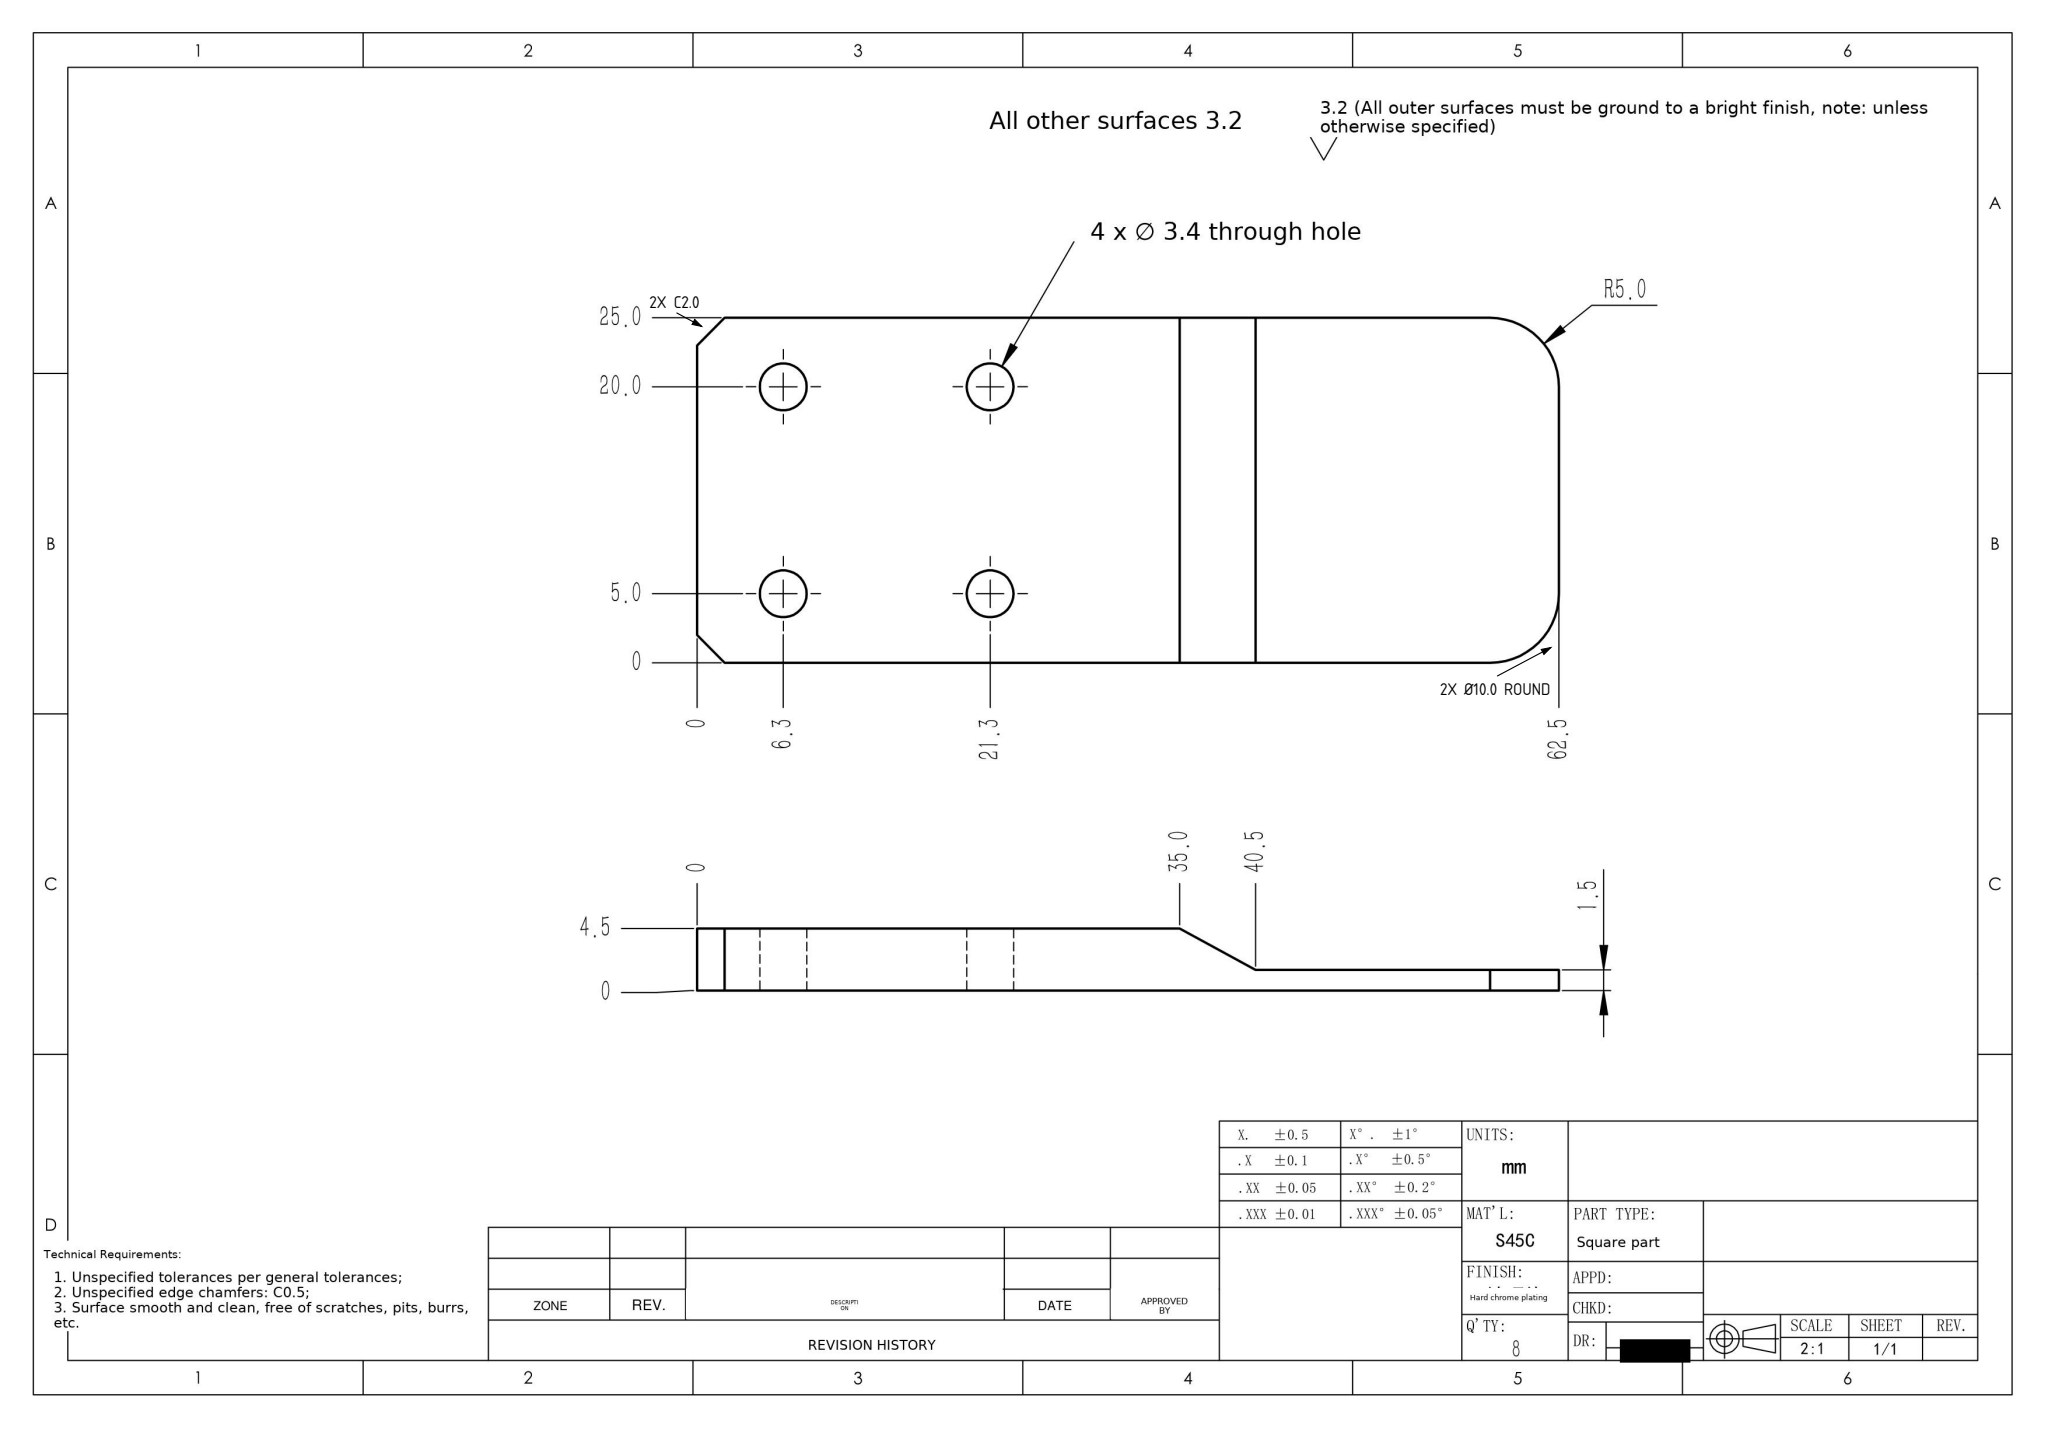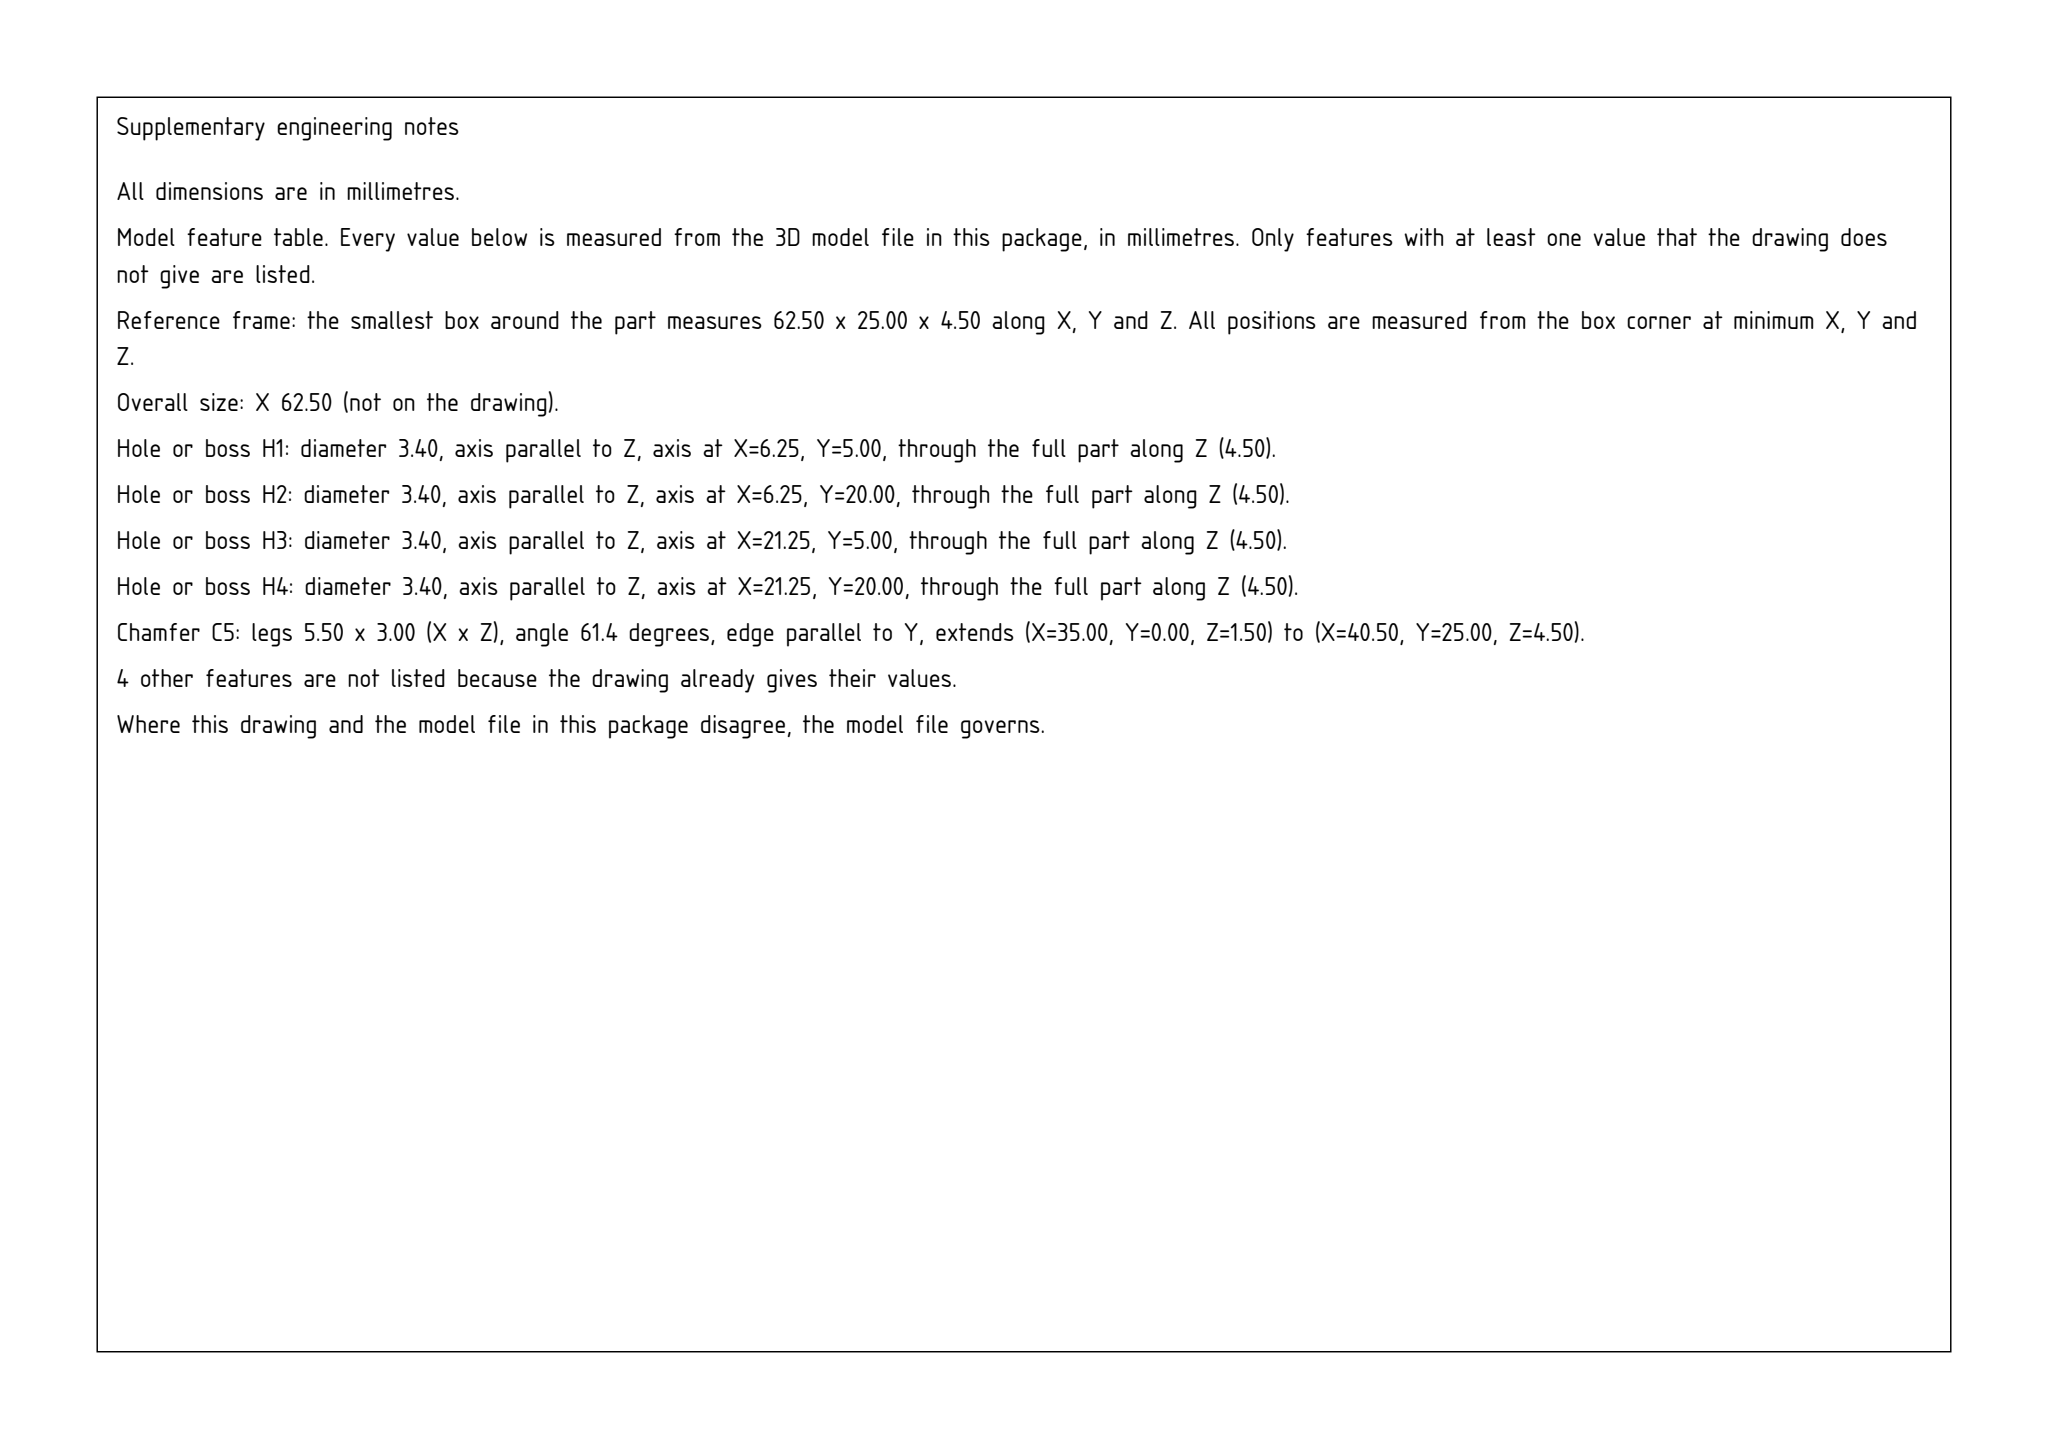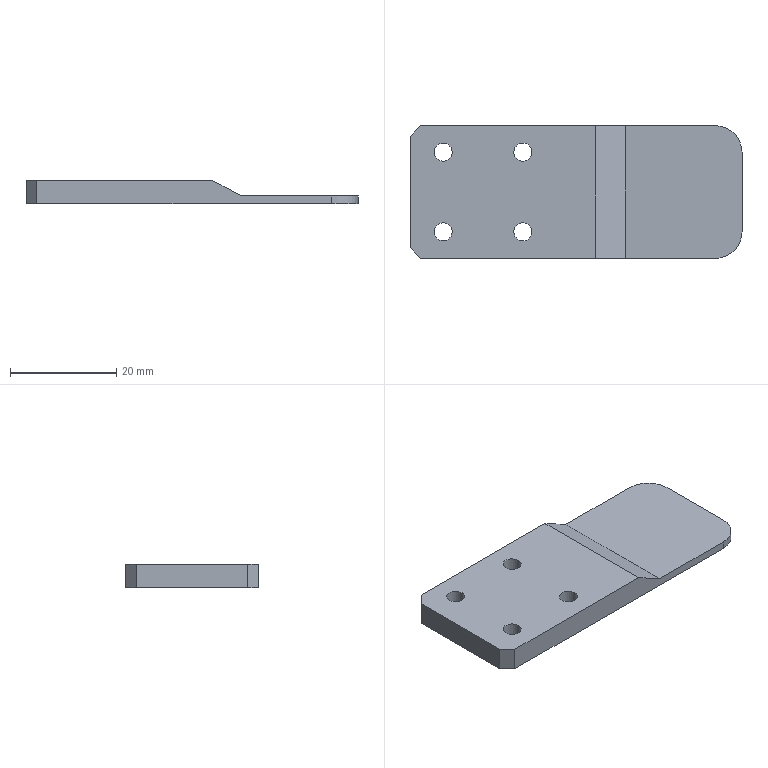Part | SolidWorks | mm | material S45C | 1 solid | 20 faces | box 62.5 x 25 x 4.5 mm | volume 4977 mm3 | cylinder 10 | plane 10 | commonest cylinder face diameters 3.4 x8 10 x2
Drawing notes:
2X Ø10.0 feature through the 1.5 thk end section, axes normal to the top face, centers at X=57.5 from the left end face and Y=5.0 and Y=20.0 from the bottom edge. | from the solid: cylinders [10.0, axis z, pos (57.5, 5.0) and (57.5, 20.0), length 1.5]
2X CHAMFER 2.0 X 45° ON LEFT END VERTICAL CORNERS (AT X=0 FACE, AT Y=0 AND Y=25.0 EDGES), FULL 4.5 THICKNESS | from the solid: inclined_planes: two faces at 45.0/45.0/90.0 deg, bbox_from [0.0,0.0,0.0] and [0.0,23.0,0.0], size [2.0,2.0,4.5]; x=0 plane extent y 2.0-23.0 confirms 2.0 legs
build123d program:
from build123d import *

# Parameters (mm, degrees)
SKETCH2_W            = 62.5
SKETCH2_H            = 25
BOSS_EXTRUDE1_DEPTH  = 4.5
CUT_EXTRUDE1_DEPTH   = 41.272
M3_CLEARANCE_HOLE1_D = 3.4
FILLET1_R            = 5
CHAMFER1_SIZE        = 2


with BuildPart() as part:
    # Sketch2 → Boss-Extrude1 (new body)
    with BuildSketch(Plane.XY):
        Rectangle(SKETCH2_W, SKETCH2_H)
    extrude(amount=BOSS_EXTRUDE1_DEPTH)

    # Sketch3 → Cut-Extrude1 (cut, through all)
    with BuildSketch(Plane.XZ.offset(12.5)):
        Polygon((31.25, 1.5), (9.25, 1.5), (3.75, 4.5), (31.25, 4.5), align=None)
    extrude(amount=-CUT_EXTRUDE1_DEPTH, mode=Mode.SUBTRACT)

    # M3 Clearance Hole1 (through all)
    with Locations(Plane(origin=(0, 0, 0), x_dir=(-1, 0, 0), z_dir=(0, 0, -1))):
        with Locations((10, -7.5), (10, 7.5), (25, 7.5), (25, -7.5)):
            Hole(M3_CLEARANCE_HOLE1_D / 2)

    # Fillet1
    fillet1_edges = [part.edges().sort_by_distance(p)[0] for p in [
        (31.25, -12.5, 0.75),
        (31.25, 12.5, 0.75),
    ]]
    fillet(fillet1_edges, radius=FILLET1_R)

    # Chamfer1
    chamfer1_edges = [part.edges().sort_by_distance(p)[0] for p in [
        (-31.25, -12.5, 2.25),
        (-31.25, 12.5, 2.25),
    ]]
    chamfer(chamfer1_edges, length=CHAMFER1_SIZE)


solid = part.part
STEP:
#1=CARTESIAN_POINT('',(-8.3,-7.5,4.5));
#2=VERTEX_POINT('',#1);
#3=CARTESIAN_POINT('',(-11.7,-7.5,4.5));
#4=VERTEX_POINT('',#3);
#5=CARTESIAN_POINT('',(-10.,-7.5,4.5));
#6=DIRECTION('',(0.,0.,-1.));
#7=DIRECTION('',(-1.,0.,0.));
#8=AXIS2_PLACEMENT_3D('',#5,#6,#7);
#9=CIRCLE('',#8,1.7);
#10=EDGE_CURVE('',#2,#4,#9,.T.);
#11=ORIENTED_EDGE('',*,*,#10,.F.);
#12=CARTESIAN_POINT('',(-8.3,-7.5,-0.));
#13=VERTEX_POINT('',#12);
#14=CARTESIAN_POINT('',(-8.3,-7.5,0.));
#15=DIRECTION('',(0.,0.,-1.));
#16=VECTOR('',#15,1000.);
#17=LINE('',#14,#16);
#18=EDGE_CURVE('',#2,#13,#17,.T.);
#19=ORIENTED_EDGE('',*,*,#18,.T.);
#20=CARTESIAN_POINT('',(-11.7,-7.5,-0.));
#21=VERTEX_POINT('',#20);
#22=CARTESIAN_POINT('',(-10.,-7.5,-0.));
#23=DIRECTION('',(0.,0.,-1.));
#24=DIRECTION('',(-1.,0.,0.));
#25=AXIS2_PLACEMENT_3D('',#22,#23,#24);
#26=CIRCLE('',#25,1.7);
#27=EDGE_CURVE('',#13,#21,#26,.T.);
#28=ORIENTED_EDGE('',*,*,#27,.T.);
#29=CARTESIAN_POINT('',(-11.7,-7.5,0.));
#30=DIRECTION('',(0.,0.,-1.));
#31=VECTOR('',#30,1000.);
#32=LINE('',#29,#31);
#33=EDGE_CURVE('',#4,#21,#32,.T.);
#34=ORIENTED_EDGE('',*,*,#33,.F.);
#35=EDGE_LOOP('',(#11,#19,#28,#34));
#36=FACE_OUTER_BOUND('',#35,.T.);
#37=CARTESIAN_POINT('',(-10.,-7.5,0.));
#38=DIRECTION('',(0.,0.,-1.));
#39=DIRECTION('',(-1.,0.,0.));
#40=AXIS2_PLACEMENT_3D('',#37,#38,#39);
#41=CYLINDRICAL_SURFACE('',#40,1.7);
#42=ADVANCED_FACE('',(#36),#41,.F.);
#43=CARTESIAN_POINT('',(-8.3,7.5,4.5));
#44=VERTEX_POINT('',#43);
#45=CARTESIAN_POINT('',(-11.7,7.5,4.5));
#46=VERTEX_POINT('',#45);
#47=CARTESIAN_POINT('',(-10.,7.5,4.5));
#48=DIRECTION('',(0.,0.,-1.));
#49=DIRECTION('',(-1.,0.,0.));
#50=AXIS2_PLACEMENT_3D('',#47,#48,#49);
#51=CIRCLE('',#50,1.7);
#52=EDGE_CURVE('',#44,#46,#51,.T.);
#53=ORIENTED_EDGE('',*,*,#52,.F.);
#54=CARTESIAN_POINT('',(-8.3,7.5,-0.));
#55=VERTEX_POINT('',#54);
#56=CARTESIAN_POINT('',(-8.3,7.5,0.));
#57=DIRECTION('',(0.,0.,-1.));
#58=VECTOR('',#57,1000.);
#59=LINE('',#56,#58);
#60=EDGE_CURVE('',#44,#55,#59,.T.);
#61=ORIENTED_EDGE('',*,*,#60,.T.);
#62=CARTESIAN_POINT('',(-11.7,7.5,-0.));
#63=VERTEX_POINT('',#62);
#64=CARTESIAN_POINT('',(-10.,7.5,-0.));
#65=DIRECTION('',(0.,0.,-1.));
#66=DIRECTION('',(-1.,0.,0.));
#67=AXIS2_PLACEMENT_3D('',#64,#65,#66);
#68=CIRCLE('',#67,1.7);
#69=EDGE_CURVE('',#55,#63,#68,.T.);
#70=ORIENTED_EDGE('',*,*,#69,.T.);
#71=CARTESIAN_POINT('',(-11.7,7.5,0.));
#72=DIRECTION('',(0.,0.,-1.));
#73=VECTOR('',#72,1000.);
#74=LINE('',#71,#73);
#75=EDGE_CURVE('',#46,#63,#74,.T.);
#76=ORIENTED_EDGE('',*,*,#75,.F.);
#77=EDGE_LOOP('',(#53,#61,#70,#76));
#78=FACE_OUTER_BOUND('',#77,.T.);
#79=CARTESIAN_POINT('',(-10.,7.5,0.));
#80=DIRECTION('',(0.,0.,-1.));
#81=DIRECTION('',(-1.,0.,0.));
#82=AXIS2_PLACEMENT_3D('',#79,#80,#81);
#83=CYLINDRICAL_SURFACE('',#82,1.7);
#84=ADVANCED_FACE('',(#78),#83,.F.);
#85=CARTESIAN_POINT('',(-23.3,7.5,4.5));
#86=VERTEX_POINT('',#85);
#87=CARTESIAN_POINT('',(-26.7,7.5,4.5));
#88=VERTEX_POINT('',#87);
#89=CARTESIAN_POINT('',(-25.,7.5,4.5));
#90=DIRECTION('',(0.,0.,-1.));
#91=DIRECTION('',(-1.,0.,0.));
#92=AXIS2_PLACEMENT_3D('',#89,#90,#91);
#93=CIRCLE('',#92,1.7);
#94=EDGE_CURVE('',#86,#88,#93,.T.);
#95=ORIENTED_EDGE('',*,*,#94,.F.);
#96=CARTESIAN_POINT('',(-23.3,7.5,-0.));
#97=VERTEX_POINT('',#96);
#98=CARTESIAN_POINT('',(-23.3,7.5,0.));
#99=DIRECTION('',(0.,0.,-1.));
#100=VECTOR('',#99,1000.);
#101=LINE('',#98,#100);
#102=EDGE_CURVE('',#86,#97,#101,.T.);
#103=ORIENTED_EDGE('',*,*,#102,.T.);
#104=CARTESIAN_POINT('',(-26.7,7.5,-0.));
#105=VERTEX_POINT('',#104);
#106=CARTESIAN_POINT('',(-25.,7.5,-0.));
#107=DIRECTION('',(0.,0.,-1.));
#108=DIRECTION('',(-1.,0.,0.));
#109=AXIS2_PLACEMENT_3D('',#106,#107,#108);
#110=CIRCLE('',#109,1.7);
#111=EDGE_CURVE('',#97,#105,#110,.T.);
#112=ORIENTED_EDGE('',*,*,#111,.T.);
#113=CARTESIAN_POINT('',(-26.7,7.5,0.));
#114=DIRECTION('',(0.,0.,-1.));
#115=VECTOR('',#114,1000.);
#116=LINE('',#113,#115);
#117=EDGE_CURVE('',#88,#105,#116,.T.);
#118=ORIENTED_EDGE('',*,*,#117,.F.);
#119=EDGE_LOOP('',(#95,#103,#112,#118));
#120=FACE_OUTER_BOUND('',#119,.T.);
#121=CARTESIAN_POINT('',(-25.,7.5,0.));
#122=DIRECTION('',(0.,0.,-1.));
#123=DIRECTION('',(-1.,0.,0.));
#124=AXIS2_PLACEMENT_3D('',#121,#122,#123);
#125=CYLINDRICAL_SURFACE('',#124,1.7);
#126=ADVANCED_FACE('',(#120),#125,.F.);
#127=CARTESIAN_POINT('',(-23.3,-7.5,4.5));
#128=VERTEX_POINT('',#127);
#129=CARTESIAN_POINT('',(-26.7,-7.5,4.5));
#130=VERTEX_POINT('',#129);
#131=CARTESIAN_POINT('',(-25.,-7.5,4.5));
#132=DIRECTION('',(0.,0.,-1.));
#133=DIRECTION('',(-1.,0.,0.));
#134=AXIS2_PLACEMENT_3D('',#131,#132,#133);
#135=CIRCLE('',#134,1.7);
#136=EDGE_CURVE('',#128,#130,#135,.T.);
#137=ORIENTED_EDGE('',*,*,#136,.F.);
#138=CARTESIAN_POINT('',(-23.3,-7.5,-0.));
#139=VERTEX_POINT('',#138);
#140=CARTESIAN_POINT('',(-23.3,-7.5,0.));
#141=DIRECTION('',(0.,0.,-1.));
#142=VECTOR('',#141,1000.);
#143=LINE('',#140,#142);
#144=EDGE_CURVE('',#128,#139,#143,.T.);
#145=ORIENTED_EDGE('',*,*,#144,.T.);
#146=CARTESIAN_POINT('',(-26.7,-7.5,-0.));
#147=VERTEX_POINT('',#146);
#148=CARTESIAN_POINT('',(-25.,-7.5,-0.));
#149=DIRECTION('',(0.,0.,-1.));
#150=DIRECTION('',(-1.,0.,0.));
#151=AXIS2_PLACEMENT_3D('',#148,#149,#150);
#152=CIRCLE('',#151,1.7);
#153=EDGE_CURVE('',#139,#147,#152,.T.);
#154=ORIENTED_EDGE('',*,*,#153,.T.);
#155=CARTESIAN_POINT('',(-26.7,-7.5,0.));
#156=DIRECTION('',(0.,0.,-1.));
#157=VECTOR('',#156,1000.);
#158=LINE('',#155,#157);
#159=EDGE_CURVE('',#130,#147,#158,.T.);
#160=ORIENTED_EDGE('',*,*,#159,.F.);
#161=EDGE_LOOP('',(#137,#145,#154,#160));
#162=FACE_OUTER_BOUND('',#161,.T.);
#163=CARTESIAN_POINT('',(-25.,-7.5,0.));
#164=DIRECTION('',(0.,0.,-1.));
#165=DIRECTION('',(-1.,0.,0.));
#166=AXIS2_PLACEMENT_3D('',#163,#164,#165);
#167=CYLINDRICAL_SURFACE('',#166,1.7);
#168=ADVANCED_FACE('',(#162),#167,.F.);
#169=CARTESIAN_POINT('',(31.25,7.5,1.5));
#170=VERTEX_POINT('',#169);
#171=CARTESIAN_POINT('',(31.25,-7.5,1.5));
#172=VERTEX_POINT('',#171);
#173=CARTESIAN_POINT('',(31.25,12.5,1.5));
#174=DIRECTION('',(0.,-1.,0.));
#175=VECTOR('',#174,1000.);
#176=LINE('',#173,#175);
#177=EDGE_CURVE('',#170,#172,#176,.T.);
#178=ORIENTED_EDGE('',*,*,#177,.T.);
#179=CARTESIAN_POINT('',(31.25,-7.5,0.));
#180=VERTEX_POINT('',#179);
#181=CARTESIAN_POINT('',(31.25,-7.5,4.5));
#182=DIRECTION('',(0.,0.,-1.));
#183=VECTOR('',#182,1000.);
#184=LINE('',#181,#183);
#185=EDGE_CURVE('',#172,#180,#184,.T.);
#186=ORIENTED_EDGE('',*,*,#185,.T.);
#187=CARTESIAN_POINT('',(31.25,7.5,0.));
#188=VERTEX_POINT('',#187);
#189=CARTESIAN_POINT('',(31.25,12.5,0.));
#190=DIRECTION('',(0.,1.,0.));
#191=VECTOR('',#190,1000.);
#192=LINE('',#189,#191);
#193=EDGE_CURVE('',#180,#188,#192,.T.);
#194=ORIENTED_EDGE('',*,*,#193,.T.);
#195=CARTESIAN_POINT('',(31.25,7.5,4.5));
#196=DIRECTION('',(0.,0.,1.));
#197=VECTOR('',#196,1000.);
#198=LINE('',#195,#197);
#199=EDGE_CURVE('',#188,#170,#198,.T.);
#200=ORIENTED_EDGE('',*,*,#199,.T.);
#201=EDGE_LOOP('',(#178,#186,#194,#200));
#202=FACE_OUTER_BOUND('',#201,.T.);
#203=CARTESIAN_POINT('',(31.25,12.5,4.5));
#204=DIRECTION('',(-1.,0.,0.));
#205=DIRECTION('',(0.,0.,1.));
#206=AXIS2_PLACEMENT_3D('',#203,#204,#205);
#207=PLANE('',#206);
#208=ADVANCED_FACE('',(#202),#207,.F.);
#209=CARTESIAN_POINT('',(26.25,12.5,0.));
#210=VERTEX_POINT('',#209);
#211=CARTESIAN_POINT('',(-29.25,12.5,0.));
#212=VERTEX_POINT('',#211);
#213=CARTESIAN_POINT('',(-31.25,12.5,0.));
#214=DIRECTION('',(-1.,0.,0.));
#215=VECTOR('',#214,1000.);
#216=LINE('',#213,#215);
#217=EDGE_CURVE('',#210,#212,#216,.T.);
#218=ORIENTED_EDGE('',*,*,#217,.T.);
#219=CARTESIAN_POINT('',(-29.25,12.5,4.5));
#220=VERTEX_POINT('',#219);
#221=CARTESIAN_POINT('',(-29.25,12.5,4.5));
#222=DIRECTION('',(0.,0.,1.));
#223=VECTOR('',#222,1000.);
#224=LINE('',#221,#223);
#225=EDGE_CURVE('',#212,#220,#224,.T.);
#226=ORIENTED_EDGE('',*,*,#225,.T.);
#227=CARTESIAN_POINT('',(3.75,12.5,4.5));
#228=VERTEX_POINT('',#227);
#229=CARTESIAN_POINT('',(-31.25,12.5,4.5));
#230=DIRECTION('',(-1.,0.,0.));
#231=VECTOR('',#230,1000.);
#232=LINE('',#229,#231);
#233=EDGE_CURVE('',#228,#220,#232,.T.);
#234=ORIENTED_EDGE('',*,*,#233,.F.);
#235=CARTESIAN_POINT('',(9.25,12.5,1.5));
#236=VERTEX_POINT('',#235);
#237=CARTESIAN_POINT('',(9.25,12.5,1.5));
#238=DIRECTION('',(0.8779,0.,-0.4789));
#239=VECTOR('',#238,1000.);
#240=LINE('',#237,#239);
#241=EDGE_CURVE('',#228,#236,#240,.T.);
#242=ORIENTED_EDGE('',*,*,#241,.T.);
#243=CARTESIAN_POINT('',(26.25,12.5,1.5));
#244=VERTEX_POINT('',#243);
#245=CARTESIAN_POINT('',(31.25,12.5,1.5));
#246=DIRECTION('',(1.,0.,0.));
#247=VECTOR('',#246,1000.);
#248=LINE('',#245,#247);
#249=EDGE_CURVE('',#236,#244,#248,.T.);
#250=ORIENTED_EDGE('',*,*,#249,.T.);
#251=CARTESIAN_POINT('',(26.25,12.5,4.5));
#252=DIRECTION('',(0.,0.,-1.));
#253=VECTOR('',#252,1000.);
#254=LINE('',#251,#253);
#255=EDGE_CURVE('',#244,#210,#254,.T.);
#256=ORIENTED_EDGE('',*,*,#255,.T.);
#257=EDGE_LOOP('',(#218,#226,#234,#242,#250,#256));
#258=FACE_OUTER_BOUND('',#257,.T.);
#259=CARTESIAN_POINT('',(-31.25,12.5,4.5));
#260=DIRECTION('',(0.,-1.,0.));
#261=DIRECTION('',(0.,0.,-1.));
#262=AXIS2_PLACEMENT_3D('',#259,#260,#261);
#263=PLANE('',#262);
#264=ADVANCED_FACE('',(#258),#263,.F.);
#265=CARTESIAN_POINT('',(-31.25,10.5,4.5));
#266=VERTEX_POINT('',#265);
#267=CARTESIAN_POINT('',(-31.25,-10.5,4.5));
#268=VERTEX_POINT('',#267);
#269=CARTESIAN_POINT('',(-31.25,12.5,4.5));
#270=DIRECTION('',(0.,-1.,0.));
#271=VECTOR('',#270,1000.);
#272=LINE('',#269,#271);
#273=EDGE_CURVE('',#266,#268,#272,.T.);
#274=ORIENTED_EDGE('',*,*,#273,.F.);
#275=CARTESIAN_POINT('',(-31.25,10.5,0.));
#276=VERTEX_POINT('',#275);
#277=CARTESIAN_POINT('',(-31.25,10.5,4.5));
#278=DIRECTION('',(0.,0.,-1.));
#279=VECTOR('',#278,1000.);
#280=LINE('',#277,#279);
#281=EDGE_CURVE('',#266,#276,#280,.T.);
#282=ORIENTED_EDGE('',*,*,#281,.T.);
#283=CARTESIAN_POINT('',(-31.25,-10.5,0.));
#284=VERTEX_POINT('',#283);
#285=CARTESIAN_POINT('',(-31.25,12.5,0.));
#286=DIRECTION('',(0.,-1.,0.));
#287=VECTOR('',#286,1000.);
#288=LINE('',#285,#287);
#289=EDGE_CURVE('',#276,#284,#288,.T.);
#290=ORIENTED_EDGE('',*,*,#289,.T.);
#291=CARTESIAN_POINT('',(-31.25,-10.5,4.5));
#292=DIRECTION('',(0.,0.,1.));
#293=VECTOR('',#292,1000.);
#294=LINE('',#291,#293);
#295=EDGE_CURVE('',#284,#268,#294,.T.);
#296=ORIENTED_EDGE('',*,*,#295,.T.);
#297=EDGE_LOOP('',(#274,#282,#290,#296));
#298=FACE_OUTER_BOUND('',#297,.T.);
#299=CARTESIAN_POINT('',(-31.25,12.5,4.5));
#300=DIRECTION('',(1.,0.,0.));
#301=DIRECTION('',(-0.,1.,0.));
#302=AXIS2_PLACEMENT_3D('',#299,#300,#301);
#303=PLANE('',#302);
#304=ADVANCED_FACE('',(#298),#303,.F.);
#305=CARTESIAN_POINT('',(-29.25,-12.5,4.5));
#306=VERTEX_POINT('',#305);
#307=CARTESIAN_POINT('',(3.75,-12.5,4.5));
#308=VERTEX_POINT('',#307);
#309=CARTESIAN_POINT('',(-31.25,-12.5,4.5));
#310=DIRECTION('',(1.,0.,0.));
#311=VECTOR('',#310,1000.);
#312=LINE('',#309,#311);
#313=EDGE_CURVE('',#306,#308,#312,.T.);
#314=ORIENTED_EDGE('',*,*,#313,.F.);
#315=CARTESIAN_POINT('',(-29.25,-12.5,0.));
#316=VERTEX_POINT('',#315);
#317=CARTESIAN_POINT('',(-29.25,-12.5,4.5));
#318=DIRECTION('',(0.,0.,-1.));
#319=VECTOR('',#318,1000.);
#320=LINE('',#317,#319);
#321=EDGE_CURVE('',#306,#316,#320,.T.);
#322=ORIENTED_EDGE('',*,*,#321,.T.);
#323=CARTESIAN_POINT('',(26.25,-12.5,0.));
#324=VERTEX_POINT('',#323);
#325=CARTESIAN_POINT('',(-31.25,-12.5,0.));
#326=DIRECTION('',(1.,0.,0.));
#327=VECTOR('',#326,1000.);
#328=LINE('',#325,#327);
#329=EDGE_CURVE('',#316,#324,#328,.T.);
#330=ORIENTED_EDGE('',*,*,#329,.T.);
#331=CARTESIAN_POINT('',(26.25,-12.5,1.5));
#332=VERTEX_POINT('',#331);
#333=CARTESIAN_POINT('',(26.25,-12.5,4.5));
#334=DIRECTION('',(0.,0.,1.));
#335=VECTOR('',#334,1000.);
#336=LINE('',#333,#335);
#337=EDGE_CURVE('',#324,#332,#336,.T.);
#338=ORIENTED_EDGE('',*,*,#337,.T.);
#339=CARTESIAN_POINT('',(9.25,-12.5,1.5));
#340=VERTEX_POINT('',#339);
#341=CARTESIAN_POINT('',(31.25,-12.5,1.5));
#342=DIRECTION('',(1.,0.,0.));
#343=VECTOR('',#342,1000.);
#344=LINE('',#341,#343);
#345=EDGE_CURVE('',#340,#332,#344,.T.);
#346=ORIENTED_EDGE('',*,*,#345,.F.);
#347=CARTESIAN_POINT('',(9.25,-12.5,1.5));
#348=DIRECTION('',(0.8779,0.,-0.4789));
#349=VECTOR('',#348,1000.);
#350=LINE('',#347,#349);
#351=EDGE_CURVE('',#308,#340,#350,.T.);
#352=ORIENTED_EDGE('',*,*,#351,.F.);
#353=EDGE_LOOP('',(#314,#322,#330,#338,#346,#352));
#354=FACE_OUTER_BOUND('',#353,.T.);
#355=CARTESIAN_POINT('',(-31.25,-12.5,4.5));
#356=DIRECTION('',(0.,1.,0.));
#357=DIRECTION('',(0.,0.,1.));
#358=AXIS2_PLACEMENT_3D('',#355,#356,#357);
#359=PLANE('',#358);
#360=ADVANCED_FACE('',(#354),#359,.F.);
#361=CARTESIAN_POINT('',(-10.,-7.5,4.5));
#362=DIRECTION('',(0.,0.,-1.));
#363=DIRECTION('',(-1.,0.,0.));
#364=AXIS2_PLACEMENT_3D('',#361,#362,#363);
#365=CIRCLE('',#364,1.7);
#366=EDGE_CURVE('',#4,#2,#365,.T.);
#367=ORIENTED_EDGE('',*,*,#366,.T.);
#368=ORIENTED_EDGE('',*,*,#10,.T.);
#369=EDGE_LOOP('',(#367,#368));
#370=FACE_BOUND('',#369,.T.);
#371=CARTESIAN_POINT('',(-10.,7.5,4.5));
#372=DIRECTION('',(0.,0.,-1.));
#373=DIRECTION('',(-1.,0.,0.));
#374=AXIS2_PLACEMENT_3D('',#371,#372,#373);
#375=CIRCLE('',#374,1.7);
#376=EDGE_CURVE('',#46,#44,#375,.T.);
#377=ORIENTED_EDGE('',*,*,#376,.T.);
#378=ORIENTED_EDGE('',*,*,#52,.T.);
#379=EDGE_LOOP('',(#377,#378));
#380=FACE_BOUND('',#379,.T.);
#381=CARTESIAN_POINT('',(-25.,7.5,4.5));
#382=DIRECTION('',(0.,0.,-1.));
#383=DIRECTION('',(-1.,0.,0.));
#384=AXIS2_PLACEMENT_3D('',#381,#382,#383);
#385=CIRCLE('',#384,1.7);
#386=EDGE_CURVE('',#88,#86,#385,.T.);
#387=ORIENTED_EDGE('',*,*,#386,.T.);
#388=ORIENTED_EDGE('',*,*,#94,.T.);
#389=EDGE_LOOP('',(#387,#388));
#390=FACE_BOUND('',#389,.T.);
#391=CARTESIAN_POINT('',(-25.,-7.5,4.5));
#392=DIRECTION('',(0.,0.,-1.));
#393=DIRECTION('',(-1.,0.,0.));
#394=AXIS2_PLACEMENT_3D('',#391,#392,#393);
#395=CIRCLE('',#394,1.7);
#396=EDGE_CURVE('',#130,#128,#395,.T.);
#397=ORIENTED_EDGE('',*,*,#396,.T.);
#398=ORIENTED_EDGE('',*,*,#136,.T.);
#399=EDGE_LOOP('',(#397,#398));
#400=FACE_BOUND('',#399,.T.);
#401=ORIENTED_EDGE('',*,*,#233,.T.);
#402=CARTESIAN_POINT('',(-20.875,20.875,4.5));
#403=DIRECTION('',(-0.7071,-0.7071,0.));
#404=VECTOR('',#403,1000.);
#405=LINE('',#402,#404);
#406=EDGE_CURVE('',#220,#266,#405,.T.);
#407=ORIENTED_EDGE('',*,*,#406,.T.);
#408=ORIENTED_EDGE('',*,*,#273,.T.);
#409=CARTESIAN_POINT('',(-20.875,-20.875,4.5));
#410=DIRECTION('',(0.7071,-0.7071,0.));
#411=VECTOR('',#410,1000.);
#412=LINE('',#409,#411);
#413=EDGE_CURVE('',#268,#306,#412,.T.);
#414=ORIENTED_EDGE('',*,*,#413,.T.);
#415=ORIENTED_EDGE('',*,*,#313,.T.);
#416=CARTESIAN_POINT('',(3.75,12.5,4.5));
#417=DIRECTION('',(0.,-1.,0.));
#418=VECTOR('',#417,1000.);
#419=LINE('',#416,#418);
#420=EDGE_CURVE('',#228,#308,#419,.T.);
#421=ORIENTED_EDGE('',*,*,#420,.F.);
#422=EDGE_LOOP('',(#401,#407,#408,#414,#415,#421));
#423=FACE_OUTER_BOUND('',#422,.T.);
#424=CARTESIAN_POINT('',(0.,0.,4.5));
#425=DIRECTION('',(0.,0.,1.));
#426=DIRECTION('',(1.,0.,0.));
#427=AXIS2_PLACEMENT_3D('',#424,#425,#426);
#428=PLANE('',#427);
#429=ADVANCED_FACE('',(#370,#380,#390,#400,#423),#428,.T.);
#430=CARTESIAN_POINT('',(-10.,-7.5,-0.));
#431=DIRECTION('',(0.,0.,-1.));
#432=DIRECTION('',(-1.,0.,0.));
#433=AXIS2_PLACEMENT_3D('',#430,#431,#432);
#434=CIRCLE('',#433,1.7);
#435=EDGE_CURVE('',#21,#13,#434,.T.);
#436=ORIENTED_EDGE('',*,*,#435,.F.);
#437=ORIENTED_EDGE('',*,*,#27,.F.);
#438=EDGE_LOOP('',(#436,#437));
#439=FACE_BOUND('',#438,.T.);
#440=CARTESIAN_POINT('',(-10.,7.5,-0.));
#441=DIRECTION('',(0.,0.,-1.));
#442=DIRECTION('',(-1.,0.,0.));
#443=AXIS2_PLACEMENT_3D('',#440,#441,#442);
#444=CIRCLE('',#443,1.7);
#445=EDGE_CURVE('',#63,#55,#444,.T.);
#446=ORIENTED_EDGE('',*,*,#445,.F.);
#447=ORIENTED_EDGE('',*,*,#69,.F.);
#448=EDGE_LOOP('',(#446,#447));
#449=FACE_BOUND('',#448,.T.);
#450=CARTESIAN_POINT('',(-25.,7.5,-0.));
#451=DIRECTION('',(0.,0.,-1.));
#452=DIRECTION('',(-1.,0.,0.));
#453=AXIS2_PLACEMENT_3D('',#450,#451,#452);
#454=CIRCLE('',#453,1.7);
#455=EDGE_CURVE('',#105,#97,#454,.T.);
#456=ORIENTED_EDGE('',*,*,#455,.F.);
#457=ORIENTED_EDGE('',*,*,#111,.F.);
#458=EDGE_LOOP('',(#456,#457));
#459=FACE_BOUND('',#458,.T.);
#460=CARTESIAN_POINT('',(-25.,-7.5,-0.));
#461=DIRECTION('',(0.,0.,-1.));
#462=DIRECTION('',(-1.,0.,0.));
#463=AXIS2_PLACEMENT_3D('',#460,#461,#462);
#464=CIRCLE('',#463,1.7);
#465=EDGE_CURVE('',#147,#139,#464,.T.);
#466=ORIENTED_EDGE('',*,*,#465,.F.);
#467=ORIENTED_EDGE('',*,*,#153,.F.);
#468=EDGE_LOOP('',(#466,#467));
#469=FACE_BOUND('',#468,.T.);
#470=ORIENTED_EDGE('',*,*,#289,.F.);
#471=CARTESIAN_POINT('',(-31.25,10.5,0.));
#472=DIRECTION('',(0.7071,0.7071,0.));
#473=VECTOR('',#472,1000.);
#474=LINE('',#471,#473);
#475=EDGE_CURVE('',#276,#212,#474,.T.);
#476=ORIENTED_EDGE('',*,*,#475,.T.);
#477=ORIENTED_EDGE('',*,*,#217,.F.);
#478=CARTESIAN_POINT('',(26.25,7.5,0.));
#479=DIRECTION('',(0.,0.,-1.));
#480=DIRECTION('',(1.,0.,0.));
#481=AXIS2_PLACEMENT_3D('',#478,#479,#480);
#482=CIRCLE('',#481,5.);
#483=EDGE_CURVE('',#210,#188,#482,.T.);
#484=ORIENTED_EDGE('',*,*,#483,.T.);
#485=ORIENTED_EDGE('',*,*,#193,.F.);
#486=CARTESIAN_POINT('',(26.25,-7.5,0.));
#487=DIRECTION('',(0.,0.,-1.));
#488=DIRECTION('',(1.,0.,0.));
#489=AXIS2_PLACEMENT_3D('',#486,#487,#488);
#490=CIRCLE('',#489,5.);
#491=EDGE_CURVE('',#180,#324,#490,.T.);
#492=ORIENTED_EDGE('',*,*,#491,.T.);
#493=ORIENTED_EDGE('',*,*,#329,.F.);
#494=CARTESIAN_POINT('',(-29.25,-12.5,0.));
#495=DIRECTION('',(-0.7071,0.7071,0.));
#496=VECTOR('',#495,1000.);
#497=LINE('',#494,#496);
#498=EDGE_CURVE('',#316,#284,#497,.T.);
#499=ORIENTED_EDGE('',*,*,#498,.T.);
#500=EDGE_LOOP('',(#470,#476,#477,#484,#485,#492,#493,#499));
#501=FACE_OUTER_BOUND('',#500,.T.);
#502=CARTESIAN_POINT('',(0.,0.,0.));
#503=DIRECTION('',(0.,0.,1.));
#504=DIRECTION('',(1.,0.,0.));
#505=AXIS2_PLACEMENT_3D('',#502,#503,#504);
#506=PLANE('',#505);
#507=ADVANCED_FACE('',(#439,#449,#459,#469,#501),#506,.F.);
#508=ORIENTED_EDGE('',*,*,#345,.T.);
#509=CARTESIAN_POINT('',(26.25,-7.5,1.5));
#510=DIRECTION('',(-0.,0.,1.));
#511=DIRECTION('',(-1.,0.,-0.));
#512=AXIS2_PLACEMENT_3D('',#509,#510,#511);
#513=CIRCLE('',#512,5.);
#514=EDGE_CURVE('',#332,#172,#513,.T.);
#515=ORIENTED_EDGE('',*,*,#514,.T.);
#516=ORIENTED_EDGE('',*,*,#177,.F.);
#517=CARTESIAN_POINT('',(26.25,7.5,1.5));
#518=DIRECTION('',(-0.,0.,1.));
#519=DIRECTION('',(-1.,0.,-0.));
#520=AXIS2_PLACEMENT_3D('',#517,#518,#519);
#521=CIRCLE('',#520,5.);
#522=EDGE_CURVE('',#170,#244,#521,.T.);
#523=ORIENTED_EDGE('',*,*,#522,.T.);
#524=ORIENTED_EDGE('',*,*,#249,.F.);
#525=CARTESIAN_POINT('',(9.25,12.5,1.5));
#526=DIRECTION('',(0.,-1.,0.));
#527=VECTOR('',#526,1000.);
#528=LINE('',#525,#527);
#529=EDGE_CURVE('',#236,#340,#528,.T.);
#530=ORIENTED_EDGE('',*,*,#529,.T.);
#531=EDGE_LOOP('',(#508,#515,#516,#523,#524,#530));
#532=FACE_OUTER_BOUND('',#531,.T.);
#533=CARTESIAN_POINT('',(31.25,12.5,1.5));
#534=DIRECTION('',(0.,0.,-1.));
#535=DIRECTION('',(-1.,0.,-0.));
#536=AXIS2_PLACEMENT_3D('',#533,#534,#535);
#537=PLANE('',#536);
#538=ADVANCED_FACE('',(#532),#537,.F.);
#539=ORIENTED_EDGE('',*,*,#351,.T.);
#540=ORIENTED_EDGE('',*,*,#529,.F.);
#541=ORIENTED_EDGE('',*,*,#241,.F.);
#542=ORIENTED_EDGE('',*,*,#420,.T.);
#543=EDGE_LOOP('',(#539,#540,#541,#542));
#544=FACE_OUTER_BOUND('',#543,.T.);
#545=CARTESIAN_POINT('',(9.25,12.5,1.5));
#546=DIRECTION('',(-0.4789,0.,-0.8779));
#547=DIRECTION('',(-0.8779,0.,0.4789));
#548=AXIS2_PLACEMENT_3D('',#545,#546,#547);
#549=PLANE('',#548);
#550=ADVANCED_FACE('',(#544),#549,.F.);
#551=ORIENTED_EDGE('',*,*,#144,.F.);
#552=ORIENTED_EDGE('',*,*,#396,.F.);
#553=ORIENTED_EDGE('',*,*,#159,.T.);
#554=ORIENTED_EDGE('',*,*,#465,.T.);
#555=EDGE_LOOP('',(#551,#552,#553,#554));
#556=FACE_OUTER_BOUND('',#555,.T.);
#557=CARTESIAN_POINT('',(-25.,-7.5,0.));
#558=DIRECTION('',(0.,0.,-1.));
#559=DIRECTION('',(-1.,0.,0.));
#560=AXIS2_PLACEMENT_3D('',#557,#558,#559);
#561=CYLINDRICAL_SURFACE('',#560,1.7);
#562=ADVANCED_FACE('',(#556),#561,.F.);
#563=ORIENTED_EDGE('',*,*,#102,.F.);
#564=ORIENTED_EDGE('',*,*,#386,.F.);
#565=ORIENTED_EDGE('',*,*,#117,.T.);
#566=ORIENTED_EDGE('',*,*,#455,.T.);
#567=EDGE_LOOP('',(#563,#564,#565,#566));
#568=FACE_OUTER_BOUND('',#567,.T.);
#569=CARTESIAN_POINT('',(-25.,7.5,0.));
#570=DIRECTION('',(0.,0.,-1.));
#571=DIRECTION('',(-1.,0.,0.));
#572=AXIS2_PLACEMENT_3D('',#569,#570,#571);
#573=CYLINDRICAL_SURFACE('',#572,1.7);
#574=ADVANCED_FACE('',(#568),#573,.F.);
#575=ORIENTED_EDGE('',*,*,#60,.F.);
#576=ORIENTED_EDGE('',*,*,#376,.F.);
#577=ORIENTED_EDGE('',*,*,#75,.T.);
#578=ORIENTED_EDGE('',*,*,#445,.T.);
#579=EDGE_LOOP('',(#575,#576,#577,#578));
#580=FACE_OUTER_BOUND('',#579,.T.);
#581=CARTESIAN_POINT('',(-10.,7.5,0.));
#582=DIRECTION('',(0.,0.,-1.));
#583=DIRECTION('',(-1.,0.,0.));
#584=AXIS2_PLACEMENT_3D('',#581,#582,#583);
#585=CYLINDRICAL_SURFACE('',#584,1.7);
#586=ADVANCED_FACE('',(#580),#585,.F.);
#587=ORIENTED_EDGE('',*,*,#18,.F.);
#588=ORIENTED_EDGE('',*,*,#366,.F.);
#589=ORIENTED_EDGE('',*,*,#33,.T.);
#590=ORIENTED_EDGE('',*,*,#435,.T.);
#591=EDGE_LOOP('',(#587,#588,#589,#590));
#592=FACE_OUTER_BOUND('',#591,.T.);
#593=CARTESIAN_POINT('',(-10.,-7.5,0.));
#594=DIRECTION('',(0.,0.,-1.));
#595=DIRECTION('',(-1.,0.,0.));
#596=AXIS2_PLACEMENT_3D('',#593,#594,#595);
#597=CYLINDRICAL_SURFACE('',#596,1.7);
#598=ADVANCED_FACE('',(#592),#597,.F.);
#599=ORIENTED_EDGE('',*,*,#514,.F.);
#600=ORIENTED_EDGE('',*,*,#337,.F.);
#601=ORIENTED_EDGE('',*,*,#491,.F.);
#602=ORIENTED_EDGE('',*,*,#185,.F.);
#603=EDGE_LOOP('',(#599,#600,#601,#602));
#604=FACE_OUTER_BOUND('',#603,.T.);
#605=CARTESIAN_POINT('',(26.25,-7.5,4.5));
#606=DIRECTION('',(0.,0.,-1.));
#607=DIRECTION('',(-1.,0.,0.));
#608=AXIS2_PLACEMENT_3D('',#605,#606,#607);
#609=CYLINDRICAL_SURFACE('',#608,5.);
#610=ADVANCED_FACE('',(#604),#609,.T.);
#611=ORIENTED_EDGE('',*,*,#522,.F.);
#612=ORIENTED_EDGE('',*,*,#199,.F.);
#613=ORIENTED_EDGE('',*,*,#483,.F.);
#614=ORIENTED_EDGE('',*,*,#255,.F.);
#615=EDGE_LOOP('',(#611,#612,#613,#614));
#616=FACE_OUTER_BOUND('',#615,.T.);
#617=CARTESIAN_POINT('',(26.25,7.5,4.5));
#618=DIRECTION('',(0.,0.,-1.));
#619=DIRECTION('',(-1.,0.,0.));
#620=AXIS2_PLACEMENT_3D('',#617,#618,#619);
#621=CYLINDRICAL_SURFACE('',#620,5.);
#622=ADVANCED_FACE('',(#616),#621,.T.);
#623=ORIENTED_EDGE('',*,*,#406,.F.);
#624=ORIENTED_EDGE('',*,*,#225,.F.);
#625=ORIENTED_EDGE('',*,*,#475,.F.);
#626=ORIENTED_EDGE('',*,*,#281,.F.);
#627=EDGE_LOOP('',(#623,#624,#625,#626));
#628=FACE_OUTER_BOUND('',#627,.T.);
#629=CARTESIAN_POINT('',(-31.25,10.5,4.5));
#630=DIRECTION('',(0.7071,-0.7071,0.));
#631=DIRECTION('',(0.,0.,-1.));
#632=AXIS2_PLACEMENT_3D('',#629,#630,#631);
#633=PLANE('',#632);
#634=ADVANCED_FACE('',(#628),#633,.F.);
#635=ORIENTED_EDGE('',*,*,#413,.F.);
#636=ORIENTED_EDGE('',*,*,#295,.F.);
#637=ORIENTED_EDGE('',*,*,#498,.F.);
#638=ORIENTED_EDGE('',*,*,#321,.F.);
#639=EDGE_LOOP('',(#635,#636,#637,#638));
#640=FACE_OUTER_BOUND('',#639,.T.);
#641=CARTESIAN_POINT('',(-29.25,-12.5,4.5));
#642=DIRECTION('',(0.7071,0.7071,0.));
#643=DIRECTION('',(0.,0.,-1.));
#644=AXIS2_PLACEMENT_3D('',#641,#642,#643);
#645=PLANE('',#644);
#646=ADVANCED_FACE('',(#640),#645,.F.);
#647=CLOSED_SHELL('',(#42,#84,#126,#168,#208,#264,#304,#360,#429,#507,#538,#550,#562,#574,#586,#598,#610,#622,#634,#646));
#648=MANIFOLD_SOLID_BREP('',#647);
#649=CARTESIAN_POINT('',(0.,0.,0.));
#650=DIRECTION('',(0.,0.,1.));
#651=DIRECTION('',(1.,0.,0.));
#652=AXIS2_PLACEMENT_3D('',#649,#650,#651);
#653=(LENGTH_UNIT()NAMED_UNIT(*)SI_UNIT(.MILLI.,.METRE.));
#654=UNCERTAINTY_MEASURE_WITH_UNIT(LENGTH_MEASURE(0.00001),#653,'','');
#655=(NAMED_UNIT(*)PLANE_ANGLE_UNIT()SI_UNIT($,.RADIAN.));
#656=(NAMED_UNIT(*)SI_UNIT($,.STERADIAN.)SOLID_ANGLE_UNIT());
#657=(GEOMETRIC_REPRESENTATION_CONTEXT(3)GLOBAL_UNCERTAINTY_ASSIGNED_CONTEXT((#654))GLOBAL_UNIT_ASSIGNED_CONTEXT((#653,#655,#656))REPRESENTATION_CONTEXT('',''));
#658=ADVANCED_BREP_SHAPE_REPRESENTATION('',(#648,#652),#657);